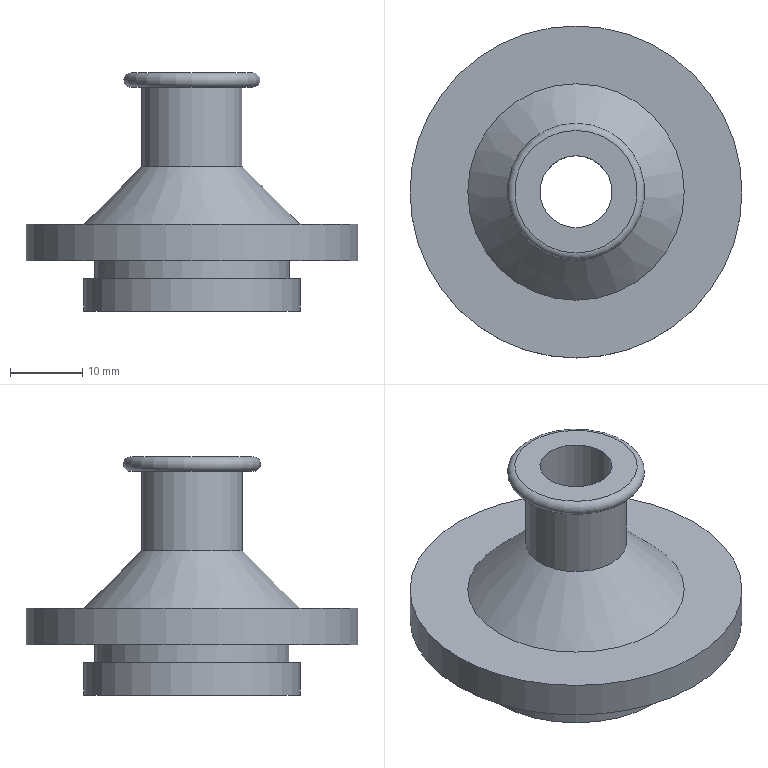Component | NX | LAMP_SOCKET | 1 solid | 15 faces | box 46 x 46 x 33 mm | volume 12206 mm3 | plane 7 | cylinder 6 | torus 1 | cone 1 | commonest cylinder face diameters 20 x1 10 x1 14 x1 46 x1 27 x1 30 x1
STEP:
#1=CARTESIAN_POINT('',(0.,0.,0.));
#2=DIRECTION('',(0.,0.,1.));
#3=DIRECTION('',(1.,0.,0.));
#4=AXIS2_PLACEMENT_3D('',#1,#2,#3);
#5=CARTESIAN_POINT('',(40.,-34.,89.));
#6=VERTEX_POINT('',#5);
#7=CARTESIAN_POINT('',(40.,-44.,89.));
#8=DIRECTION('',(0.,0.,-1.));
#9=DIRECTION('',(0.,1.,0.));
#10=AXIS2_PLACEMENT_3D('',#7,#8,#9);
#11=CIRCLE('',#10,10.);
#12=CARTESIAN_POINT('',(40.,-59.,89.));
#13=DIRECTION('',(0.,0.,1.));
#14=DIRECTION('',(0.,-1.,0.));
#15=AXIS2_PLACEMENT_3D('',#12,#13,#14);
#16=PLANE('',#15);
#17=CARTESIAN_POINT('',(-25.,0.));
#18=CARTESIAN_POINT('',(-25.,17.321));
#19=CARTESIAN_POINT('',(-10.,8.66));
#20=CARTESIAN_POINT('',(5.,0.));
#21=CARTESIAN_POINT('',(-10.,-8.66));
#22=CARTESIAN_POINT('',(-25.,-17.321));
#23=CARTESIAN_POINT('',(-25.,0.));
#24=(BOUNDED_CURVE()B_SPLINE_CURVE(2,(#17,#18,#19,#20,#21,#22,#23),.UNSPECIFIED.,.T.,.F.)B_SPLINE_CURVE_WITH_KNOTS((1,2,2,2,2,1),(-2.094,0.,2.094,4.189,6.283,8.378),.UNSPECIFIED.)CURVE()GEOMETRIC_REPRESENTATION_ITEM()RATIONAL_B_SPLINE_CURVE((1.,0.5,1.,0.5,1.,0.5,1.))REPRESENTATION_ITEM(''));
#25=(GEOMETRIC_REPRESENTATION_CONTEXT(2)PARAMETRIC_REPRESENTATION_CONTEXT()REPRESENTATION_CONTEXT('',''));
#26=DEFINITIONAL_REPRESENTATION('',(#24),#25);
#27=PCURVE('',#16,#26);
#28=CARTESIAN_POINT('',(40.,-44.,89.));
#29=DIRECTION('',(0.,0.,-1.));
#30=DIRECTION('',(0.,1.,0.));
#31=AXIS2_PLACEMENT_3D('',#28,#29,#30);
#32=CYLINDRICAL_SURFACE('',#31,10.);
#33=CARTESIAN_POINT('',(0.,0.));
#34=DIRECTION('',(1.,0.));
#35=VECTOR('',#34,1.);
#36=LINE('',#33,#35);
#37=(GEOMETRIC_REPRESENTATION_CONTEXT(2)PARAMETRIC_REPRESENTATION_CONTEXT()REPRESENTATION_CONTEXT('',''));
#38=DEFINITIONAL_REPRESENTATION('',(#36),#37);
#39=PCURVE('',#32,#38);
#40=SURFACE_CURVE('',#11,(#27,#39),.PCURVE_S1.);
#41=EDGE_CURVE('',#6,#6,#40,.T.);
#42=ORIENTED_EDGE('',*,*,#41,.F.);
#43=EDGE_LOOP('',(#42));
#44=FACE_BOUND('',#43,.T.);
#45=CARTESIAN_POINT('',(40.,-29.,89.));
#46=VERTEX_POINT('',#45);
#47=CARTESIAN_POINT('',(40.,-44.,89.));
#48=DIRECTION('',(0.,0.,-1.));
#49=DIRECTION('',(0.,1.,0.));
#50=AXIS2_PLACEMENT_3D('',#47,#48,#49);
#51=CIRCLE('',#50,15.);
#52=CARTESIAN_POINT('',(-30.,0.));
#53=CARTESIAN_POINT('',(-30.,25.981));
#54=CARTESIAN_POINT('',(-7.5,12.99));
#55=CARTESIAN_POINT('',(15.,0.));
#56=CARTESIAN_POINT('',(-7.5,-12.99));
#57=CARTESIAN_POINT('',(-30.,-25.981));
#58=CARTESIAN_POINT('',(-30.,0.));
#59=(BOUNDED_CURVE()B_SPLINE_CURVE(2,(#52,#53,#54,#55,#56,#57,#58),.UNSPECIFIED.,.T.,.F.)B_SPLINE_CURVE_WITH_KNOTS((1,2,2,2,2,1),(-2.094,0.,2.094,4.189,6.283,8.378),.UNSPECIFIED.)CURVE()GEOMETRIC_REPRESENTATION_ITEM()RATIONAL_B_SPLINE_CURVE((1.,0.5,1.,0.5,1.,0.5,1.))REPRESENTATION_ITEM(''));
#60=(GEOMETRIC_REPRESENTATION_CONTEXT(2)PARAMETRIC_REPRESENTATION_CONTEXT()REPRESENTATION_CONTEXT('',''));
#61=DEFINITIONAL_REPRESENTATION('',(#59),#60);
#62=PCURVE('',#16,#61);
#63=CARTESIAN_POINT('',(40.,-44.,89.));
#64=DIRECTION('',(0.,0.,-1.));
#65=DIRECTION('',(0.,1.,0.));
#66=AXIS2_PLACEMENT_3D('',#63,#64,#65);
#67=CYLINDRICAL_SURFACE('',#66,15.);
#68=CARTESIAN_POINT('',(0.,0.));
#69=DIRECTION('',(1.,0.));
#70=VECTOR('',#69,1.);
#71=LINE('',#68,#70);
#72=(GEOMETRIC_REPRESENTATION_CONTEXT(2)PARAMETRIC_REPRESENTATION_CONTEXT()REPRESENTATION_CONTEXT('',''));
#73=DEFINITIONAL_REPRESENTATION('',(#71),#72);
#74=PCURVE('',#67,#73);
#75=SURFACE_CURVE('',#51,(#62,#74),.PCURVE_S1.);
#76=EDGE_CURVE('',#46,#46,#75,.T.);
#77=ORIENTED_EDGE('',*,*,#76,.T.);
#78=EDGE_LOOP('',(#77));
#79=FACE_BOUND('',#78,.T.);
#80=ADVANCED_FACE('',(#44,#79),#16,.F.);
#81=CARTESIAN_POINT('',(40.,-34.,104.));
#82=VERTEX_POINT('',#81);
#83=CARTESIAN_POINT('',(40.,-44.,104.));
#84=DIRECTION('',(0.,0.,-1.));
#85=DIRECTION('',(0.,1.,0.));
#86=AXIS2_PLACEMENT_3D('',#83,#84,#85);
#87=CIRCLE('',#86,10.);
#88=CARTESIAN_POINT('',(0.,-15.));
#89=DIRECTION('',(1.,0.));
#90=VECTOR('',#89,1.);
#91=LINE('',#88,#90);
#92=(GEOMETRIC_REPRESENTATION_CONTEXT(2)PARAMETRIC_REPRESENTATION_CONTEXT()REPRESENTATION_CONTEXT('',''));
#93=DEFINITIONAL_REPRESENTATION('',(#91),#92);
#94=PCURVE('',#32,#93);
#95=CARTESIAN_POINT('',(40.,-54.,104.));
#96=DIRECTION('',(0.,0.,1.));
#97=DIRECTION('',(0.,-1.,0.));
#98=AXIS2_PLACEMENT_3D('',#95,#96,#97);
#99=PLANE('',#98);
#100=CARTESIAN_POINT('',(-20.,0.));
#101=CARTESIAN_POINT('',(-20.,17.321));
#102=CARTESIAN_POINT('',(-5.,8.66));
#103=CARTESIAN_POINT('',(10.,0.));
#104=CARTESIAN_POINT('',(-5.,-8.66));
#105=CARTESIAN_POINT('',(-20.,-17.321));
#106=CARTESIAN_POINT('',(-20.,0.));
#107=(BOUNDED_CURVE()B_SPLINE_CURVE(2,(#100,#101,#102,#103,#104,#105,#106),.UNSPECIFIED.,.T.,.F.)B_SPLINE_CURVE_WITH_KNOTS((1,2,2,2,2,1),(-2.094,0.,2.094,4.189,6.283,8.378),.UNSPECIFIED.)CURVE()GEOMETRIC_REPRESENTATION_ITEM()RATIONAL_B_SPLINE_CURVE((1.,0.5,1.,0.5,1.,0.5,1.))REPRESENTATION_ITEM(''));
#108=(GEOMETRIC_REPRESENTATION_CONTEXT(2)PARAMETRIC_REPRESENTATION_CONTEXT()REPRESENTATION_CONTEXT('',''));
#109=DEFINITIONAL_REPRESENTATION('',(#107),#108);
#110=PCURVE('',#99,#109);
#111=SURFACE_CURVE('',#87,(#94,#110),.PCURVE_S1.);
#112=EDGE_CURVE('',#82,#82,#111,.T.);
#113=ORIENTED_EDGE('',*,*,#112,.T.);
#114=CARTESIAN_POINT('',(40.,-34.,104.));
#115=CARTESIAN_POINT('',(40.,-34.,89.));
#116=B_SPLINE_CURVE_WITH_KNOTS('',1,(#114,#115),.UNSPECIFIED.,.F.,.F.,(2,2),(-15.,0.),.PIECEWISE_BEZIER_KNOTS.);
#117=CARTESIAN_POINT('',(6.283,0.));
#118=DIRECTION('',(0.,1.));
#119=VECTOR('',#118,1.);
#120=LINE('',#117,#119);
#121=(GEOMETRIC_REPRESENTATION_CONTEXT(2)PARAMETRIC_REPRESENTATION_CONTEXT()REPRESENTATION_CONTEXT('',''));
#122=DEFINITIONAL_REPRESENTATION('',(#120),#121);
#123=PCURVE('',#32,#122);
#124=CARTESIAN_POINT('',(0.,0.));
#125=DIRECTION('',(0.,1.));
#126=VECTOR('',#125,1.);
#127=LINE('',#124,#126);
#128=(GEOMETRIC_REPRESENTATION_CONTEXT(2)PARAMETRIC_REPRESENTATION_CONTEXT()REPRESENTATION_CONTEXT('',''));
#129=DEFINITIONAL_REPRESENTATION('',(#127),#128);
#130=PCURVE('',#32,#129);
#131=SEAM_CURVE('',#116,(#123,#130),.PCURVE_S1.);
#132=EDGE_CURVE('',#82,#6,#131,.T.);
#133=ORIENTED_EDGE('',*,*,#132,.T.);
#134=ORIENTED_EDGE('',*,*,#41,.F.);
#135=ORIENTED_EDGE('',*,*,#132,.F.);
#136=EDGE_LOOP('',(#113,#133,#134,#135));
#137=FACE_BOUND('',#136,.F.);
#138=ADVANCED_FACE('',(#137),#32,.F.);
#139=CARTESIAN_POINT('',(40.,-39.,104.));
#140=VERTEX_POINT('',#139);
#141=CARTESIAN_POINT('',(40.,-44.,104.));
#142=DIRECTION('',(0.,0.,-1.));
#143=DIRECTION('',(0.,1.,0.));
#144=AXIS2_PLACEMENT_3D('',#141,#142,#143);
#145=CIRCLE('',#144,5.);
#146=CARTESIAN_POINT('',(-15.,0.));
#147=CARTESIAN_POINT('',(-15.,8.66));
#148=CARTESIAN_POINT('',(-7.5,4.33));
#149=CARTESIAN_POINT('',(-0.,0.));
#150=CARTESIAN_POINT('',(-7.5,-4.33));
#151=CARTESIAN_POINT('',(-15.,-8.66));
#152=CARTESIAN_POINT('',(-15.,0.));
#153=(BOUNDED_CURVE()B_SPLINE_CURVE(2,(#146,#147,#148,#149,#150,#151,#152),.UNSPECIFIED.,.T.,.F.)B_SPLINE_CURVE_WITH_KNOTS((1,2,2,2,2,1),(-2.094,0.,2.094,4.189,6.283,8.378),.UNSPECIFIED.)CURVE()GEOMETRIC_REPRESENTATION_ITEM()RATIONAL_B_SPLINE_CURVE((1.,0.5,1.,0.5,1.,0.5,1.))REPRESENTATION_ITEM(''));
#154=(GEOMETRIC_REPRESENTATION_CONTEXT(2)PARAMETRIC_REPRESENTATION_CONTEXT()REPRESENTATION_CONTEXT('',''));
#155=DEFINITIONAL_REPRESENTATION('',(#153),#154);
#156=PCURVE('',#99,#155);
#157=CARTESIAN_POINT('',(40.,-44.,89.));
#158=DIRECTION('',(0.,0.,-1.));
#159=DIRECTION('',(0.,1.,0.));
#160=AXIS2_PLACEMENT_3D('',#157,#158,#159);
#161=CYLINDRICAL_SURFACE('',#160,5.);
#162=CARTESIAN_POINT('',(0.,-15.));
#163=DIRECTION('',(1.,0.));
#164=VECTOR('',#163,1.);
#165=LINE('',#162,#164);
#166=(GEOMETRIC_REPRESENTATION_CONTEXT(2)PARAMETRIC_REPRESENTATION_CONTEXT()REPRESENTATION_CONTEXT('',''));
#167=DEFINITIONAL_REPRESENTATION('',(#165),#166);
#168=PCURVE('',#161,#167);
#169=SURFACE_CURVE('',#145,(#156,#168),.PCURVE_S1.);
#170=EDGE_CURVE('',#140,#140,#169,.T.);
#171=ORIENTED_EDGE('',*,*,#170,.F.);
#172=EDGE_LOOP('',(#171));
#173=FACE_BOUND('',#172,.T.);
#174=ORIENTED_EDGE('',*,*,#112,.T.);
#175=EDGE_LOOP('',(#174));
#176=FACE_BOUND('',#175,.T.);
#177=ADVANCED_FACE('',(#173,#176),#99,.F.);
#178=CARTESIAN_POINT('',(40.,-39.,122.));
#179=VERTEX_POINT('',#178);
#180=CARTESIAN_POINT('',(40.,-44.,122.));
#181=DIRECTION('',(0.,0.,-1.));
#182=DIRECTION('',(0.,1.,0.));
#183=AXIS2_PLACEMENT_3D('',#180,#181,#182);
#184=CIRCLE('',#183,5.);
#185=CARTESIAN_POINT('',(0.,-33.));
#186=DIRECTION('',(1.,0.));
#187=VECTOR('',#186,1.);
#188=LINE('',#185,#187);
#189=(GEOMETRIC_REPRESENTATION_CONTEXT(2)PARAMETRIC_REPRESENTATION_CONTEXT()REPRESENTATION_CONTEXT('',''));
#190=DEFINITIONAL_REPRESENTATION('',(#188),#189);
#191=PCURVE('',#161,#190);
#192=CARTESIAN_POINT('',(40.,-49.,122.));
#193=DIRECTION('',(0.,0.,-1.));
#194=DIRECTION('',(0.,1.,0.));
#195=AXIS2_PLACEMENT_3D('',#192,#193,#194);
#196=PLANE('',#195);
#197=CARTESIAN_POINT('',(5.,0.));
#198=DIRECTION('',(1.,0.));
#199=AXIS2_PLACEMENT_2D('',#197,#198);
#200=CIRCLE('',#199,5.);
#201=(GEOMETRIC_REPRESENTATION_CONTEXT(2)PARAMETRIC_REPRESENTATION_CONTEXT()REPRESENTATION_CONTEXT('',''));
#202=DEFINITIONAL_REPRESENTATION('',(#200),#201);
#203=PCURVE('',#196,#202);
#204=SURFACE_CURVE('',#184,(#191,#203),.PCURVE_S1.);
#205=EDGE_CURVE('',#179,#179,#204,.T.);
#206=ORIENTED_EDGE('',*,*,#205,.T.);
#207=CARTESIAN_POINT('',(40.,-39.,122.));
#208=CARTESIAN_POINT('',(40.,-39.,104.));
#209=B_SPLINE_CURVE_WITH_KNOTS('',1,(#207,#208),.UNSPECIFIED.,.F.,.F.,(2,2),(-33.,-15.),.PIECEWISE_BEZIER_KNOTS.);
#210=CARTESIAN_POINT('',(6.283,0.));
#211=DIRECTION('',(0.,1.));
#212=VECTOR('',#211,1.);
#213=LINE('',#210,#212);
#214=(GEOMETRIC_REPRESENTATION_CONTEXT(2)PARAMETRIC_REPRESENTATION_CONTEXT()REPRESENTATION_CONTEXT('',''));
#215=DEFINITIONAL_REPRESENTATION('',(#213),#214);
#216=PCURVE('',#161,#215);
#217=CARTESIAN_POINT('',(0.,0.));
#218=DIRECTION('',(0.,1.));
#219=VECTOR('',#218,1.);
#220=LINE('',#217,#219);
#221=(GEOMETRIC_REPRESENTATION_CONTEXT(2)PARAMETRIC_REPRESENTATION_CONTEXT()REPRESENTATION_CONTEXT('',''));
#222=DEFINITIONAL_REPRESENTATION('',(#220),#221);
#223=PCURVE('',#161,#222);
#224=SEAM_CURVE('',#209,(#216,#223),.PCURVE_S1.);
#225=EDGE_CURVE('',#179,#140,#224,.T.);
#226=ORIENTED_EDGE('',*,*,#225,.T.);
#227=ORIENTED_EDGE('',*,*,#170,.F.);
#228=ORIENTED_EDGE('',*,*,#225,.F.);
#229=EDGE_LOOP('',(#206,#226,#227,#228));
#230=FACE_BOUND('',#229,.F.);
#231=ADVANCED_FACE('',(#230),#161,.F.);
#232=CARTESIAN_POINT('',(40.,-35.5,122.));
#233=VERTEX_POINT('',#232);
#234=CARTESIAN_POINT('',(40.,-44.,122.));
#235=DIRECTION('',(0.,0.,-1.));
#236=DIRECTION('',(0.,1.,0.));
#237=AXIS2_PLACEMENT_3D('',#234,#235,#236);
#238=CIRCLE('',#237,8.5);
#239=CARTESIAN_POINT('',(5.,0.));
#240=DIRECTION('',(1.,0.));
#241=AXIS2_PLACEMENT_2D('',#239,#240);
#242=CIRCLE('',#241,8.5);
#243=(GEOMETRIC_REPRESENTATION_CONTEXT(2)PARAMETRIC_REPRESENTATION_CONTEXT()REPRESENTATION_CONTEXT('',''));
#244=DEFINITIONAL_REPRESENTATION('',(#242),#243);
#245=PCURVE('',#196,#244);
#246=CARTESIAN_POINT('',(40.,-44.,121.));
#247=DIRECTION('',(0.,0.,-1.));
#248=DIRECTION('',(0.,1.,0.));
#249=AXIS2_PLACEMENT_3D('',#246,#247,#248);
#250=TOROIDAL_SURFACE('',#249,8.5,1.);
#251=CARTESIAN_POINT('',(0.,4.712));
#252=DIRECTION('',(1.,0.));
#253=VECTOR('',#252,1.);
#254=LINE('',#251,#253);
#255=(GEOMETRIC_REPRESENTATION_CONTEXT(2)PARAMETRIC_REPRESENTATION_CONTEXT()REPRESENTATION_CONTEXT('',''));
#256=DEFINITIONAL_REPRESENTATION('',(#254),#255);
#257=PCURVE('',#250,#256);
#258=SURFACE_CURVE('',#238,(#245,#257),.PCURVE_S1.);
#259=EDGE_CURVE('',#233,#233,#258,.T.);
#260=ORIENTED_EDGE('',*,*,#259,.F.);
#261=EDGE_LOOP('',(#260));
#262=FACE_BOUND('',#261,.T.);
#263=ORIENTED_EDGE('',*,*,#205,.T.);
#264=EDGE_LOOP('',(#263));
#265=FACE_BOUND('',#264,.T.);
#266=ADVANCED_FACE('',(#262,#265),#196,.F.);
#267=CARTESIAN_POINT('',(40.,-35.5,120.));
#268=VERTEX_POINT('',#267);
#269=CARTESIAN_POINT('',(40.,-44.,120.));
#270=DIRECTION('',(0.,0.,-1.));
#271=DIRECTION('',(0.,1.,0.));
#272=AXIS2_PLACEMENT_3D('',#269,#270,#271);
#273=CIRCLE('',#272,8.5);
#274=CARTESIAN_POINT('',(0.,7.854));
#275=DIRECTION('',(1.,0.));
#276=VECTOR('',#275,1.);
#277=LINE('',#274,#276);
#278=(GEOMETRIC_REPRESENTATION_CONTEXT(2)PARAMETRIC_REPRESENTATION_CONTEXT()REPRESENTATION_CONTEXT('',''));
#279=DEFINITIONAL_REPRESENTATION('',(#277),#278);
#280=PCURVE('',#250,#279);
#281=CARTESIAN_POINT('',(40.,-52.5,120.));
#282=DIRECTION('',(0.,0.,1.));
#283=DIRECTION('',(0.,-1.,0.));
#284=AXIS2_PLACEMENT_3D('',#281,#282,#283);
#285=PLANE('',#284);
#286=CARTESIAN_POINT('',(-17.,0.));
#287=CARTESIAN_POINT('',(-17.,14.722));
#288=CARTESIAN_POINT('',(-4.25,7.361));
#289=CARTESIAN_POINT('',(8.5,0.));
#290=CARTESIAN_POINT('',(-4.25,-7.361));
#291=CARTESIAN_POINT('',(-17.,-14.722));
#292=CARTESIAN_POINT('',(-17.,0.));
#293=(BOUNDED_CURVE()B_SPLINE_CURVE(2,(#286,#287,#288,#289,#290,#291,#292),.UNSPECIFIED.,.T.,.F.)B_SPLINE_CURVE_WITH_KNOTS((1,2,2,2,2,1),(-2.094,0.,2.094,4.189,6.283,8.378),.UNSPECIFIED.)CURVE()GEOMETRIC_REPRESENTATION_ITEM()RATIONAL_B_SPLINE_CURVE((1.,0.5,1.,0.5,1.,0.5,1.))REPRESENTATION_ITEM(''));
#294=(GEOMETRIC_REPRESENTATION_CONTEXT(2)PARAMETRIC_REPRESENTATION_CONTEXT()REPRESENTATION_CONTEXT('',''));
#295=DEFINITIONAL_REPRESENTATION('',(#293),#294);
#296=PCURVE('',#285,#295);
#297=SURFACE_CURVE('',#273,(#280,#296),.PCURVE_S1.);
#298=EDGE_CURVE('',#268,#268,#297,.T.);
#299=ORIENTED_EDGE('',*,*,#298,.F.);
#300=CARTESIAN_POINT('',(40.,-35.5,122.));
#301=CARTESIAN_POINT('',(40.,-35.107,122.));
#302=CARTESIAN_POINT('',(40.,-34.715,121.824));
#303=CARTESIAN_POINT('',(40.,-34.414,121.471));
#304=CARTESIAN_POINT('',(40.,-34.298,121.));
#305=CARTESIAN_POINT('',(40.,-34.414,120.529));
#306=CARTESIAN_POINT('',(40.,-34.715,120.176));
#307=CARTESIAN_POINT('',(40.,-35.107,120.));
#308=CARTESIAN_POINT('',(40.,-35.5,120.));
#309=B_SPLINE_CURVE_WITH_KNOTS('',8,(#300,#301,#302,#303,#304,#305,#306,#307,#308),.UNSPECIFIED.,.F.,.F.,(9,9),(-1.571,1.571),.PIECEWISE_BEZIER_KNOTS.);
#310=CARTESIAN_POINT('',(0.,6.283));
#311=DIRECTION('',(0.,1.));
#312=VECTOR('',#311,1.);
#313=LINE('',#310,#312);
#314=(GEOMETRIC_REPRESENTATION_CONTEXT(2)PARAMETRIC_REPRESENTATION_CONTEXT()REPRESENTATION_CONTEXT('',''));
#315=DEFINITIONAL_REPRESENTATION('',(#313),#314);
#316=PCURVE('',#250,#315);
#317=CARTESIAN_POINT('',(6.283,6.283));
#318=DIRECTION('',(0.,1.));
#319=VECTOR('',#318,1.);
#320=LINE('',#317,#319);
#321=(GEOMETRIC_REPRESENTATION_CONTEXT(2)PARAMETRIC_REPRESENTATION_CONTEXT()REPRESENTATION_CONTEXT('',''));
#322=DEFINITIONAL_REPRESENTATION('',(#320),#321);
#323=PCURVE('',#250,#322);
#324=SEAM_CURVE('',#309,(#316,#323),.PCURVE_S1.);
#325=EDGE_CURVE('',#233,#268,#324,.T.);
#326=ORIENTED_EDGE('',*,*,#325,.F.);
#327=ORIENTED_EDGE('',*,*,#259,.T.);
#328=ORIENTED_EDGE('',*,*,#325,.T.);
#329=EDGE_LOOP('',(#299,#326,#327,#328));
#330=FACE_BOUND('',#329,.T.);
#331=ADVANCED_FACE('',(#330),#250,.T.);
#332=CARTESIAN_POINT('',(40.,-37.,120.));
#333=VERTEX_POINT('',#332);
#334=CARTESIAN_POINT('',(40.,-44.,120.));
#335=DIRECTION('',(0.,0.,-1.));
#336=DIRECTION('',(0.,1.,0.));
#337=AXIS2_PLACEMENT_3D('',#334,#335,#336);
#338=CIRCLE('',#337,7.);
#339=CARTESIAN_POINT('',(-15.5,0.));
#340=CARTESIAN_POINT('',(-15.5,12.124));
#341=CARTESIAN_POINT('',(-5.,6.062));
#342=CARTESIAN_POINT('',(5.5,0.));
#343=CARTESIAN_POINT('',(-5.,-6.062));
#344=CARTESIAN_POINT('',(-15.5,-12.124));
#345=CARTESIAN_POINT('',(-15.5,0.));
#346=(BOUNDED_CURVE()B_SPLINE_CURVE(2,(#339,#340,#341,#342,#343,#344,#345),.UNSPECIFIED.,.T.,.F.)B_SPLINE_CURVE_WITH_KNOTS((1,2,2,2,2,1),(-2.094,0.,2.094,4.189,6.283,8.378),.UNSPECIFIED.)CURVE()GEOMETRIC_REPRESENTATION_ITEM()RATIONAL_B_SPLINE_CURVE((1.,0.5,1.,0.5,1.,0.5,1.))REPRESENTATION_ITEM(''));
#347=(GEOMETRIC_REPRESENTATION_CONTEXT(2)PARAMETRIC_REPRESENTATION_CONTEXT()REPRESENTATION_CONTEXT('',''));
#348=DEFINITIONAL_REPRESENTATION('',(#346),#347);
#349=PCURVE('',#285,#348);
#350=CARTESIAN_POINT('',(40.,-44.,89.));
#351=DIRECTION('',(0.,0.,-1.));
#352=DIRECTION('',(0.,1.,0.));
#353=AXIS2_PLACEMENT_3D('',#350,#351,#352);
#354=CYLINDRICAL_SURFACE('',#353,7.);
#355=CARTESIAN_POINT('',(0.,-31.));
#356=DIRECTION('',(1.,0.));
#357=VECTOR('',#356,1.);
#358=LINE('',#355,#357);
#359=(GEOMETRIC_REPRESENTATION_CONTEXT(2)PARAMETRIC_REPRESENTATION_CONTEXT()REPRESENTATION_CONTEXT('',''));
#360=DEFINITIONAL_REPRESENTATION('',(#358),#359);
#361=PCURVE('',#354,#360);
#362=SURFACE_CURVE('',#338,(#349,#361),.PCURVE_S1.);
#363=EDGE_CURVE('',#333,#333,#362,.T.);
#364=ORIENTED_EDGE('',*,*,#363,.F.);
#365=EDGE_LOOP('',(#364));
#366=FACE_BOUND('',#365,.T.);
#367=ORIENTED_EDGE('',*,*,#298,.T.);
#368=EDGE_LOOP('',(#367));
#369=FACE_BOUND('',#368,.T.);
#370=ADVANCED_FACE('',(#366,#369),#285,.F.);
#371=CARTESIAN_POINT('',(40.,-37.,109.));
#372=VERTEX_POINT('',#371);
#373=CARTESIAN_POINT('',(40.,-44.,109.));
#374=DIRECTION('',(0.,0.,-1.));
#375=DIRECTION('',(0.,1.,0.));
#376=AXIS2_PLACEMENT_3D('',#373,#374,#375);
#377=CIRCLE('',#376,7.);
#378=CARTESIAN_POINT('',(0.,-20.));
#379=DIRECTION('',(1.,0.));
#380=VECTOR('',#379,1.);
#381=LINE('',#378,#380);
#382=(GEOMETRIC_REPRESENTATION_CONTEXT(2)PARAMETRIC_REPRESENTATION_CONTEXT()REPRESENTATION_CONTEXT('',''));
#383=DEFINITIONAL_REPRESENTATION('',(#381),#382);
#384=PCURVE('',#354,#383);
#385=CARTESIAN_POINT('',(40.,-44.,109.));
#386=DIRECTION('',(0.,0.,-1.));
#387=DIRECTION('',(0.,1.,0.));
#388=AXIS2_PLACEMENT_3D('',#385,#386,#387);
#389=CONICAL_SURFACE('',#388,7.,0.7854);
#390=CARTESIAN_POINT('',(0.,0.));
#391=DIRECTION('',(1.,0.));
#392=VECTOR('',#391,1.);
#393=LINE('',#390,#392);
#394=(GEOMETRIC_REPRESENTATION_CONTEXT(2)PARAMETRIC_REPRESENTATION_CONTEXT()REPRESENTATION_CONTEXT('',''));
#395=DEFINITIONAL_REPRESENTATION('',(#393),#394);
#396=PCURVE('',#389,#395);
#397=SURFACE_CURVE('',#377,(#384,#396),.PCURVE_S1.);
#398=EDGE_CURVE('',#372,#372,#397,.T.);
#399=ORIENTED_EDGE('',*,*,#398,.F.);
#400=CARTESIAN_POINT('',(40.,-37.,120.));
#401=CARTESIAN_POINT('',(40.,-37.,109.));
#402=B_SPLINE_CURVE_WITH_KNOTS('',1,(#400,#401),.UNSPECIFIED.,.F.,.F.,(2,2),(-31.,-20.),.PIECEWISE_BEZIER_KNOTS.);
#403=CARTESIAN_POINT('',(0.,0.));
#404=DIRECTION('',(0.,1.));
#405=VECTOR('',#404,1.);
#406=LINE('',#403,#405);
#407=(GEOMETRIC_REPRESENTATION_CONTEXT(2)PARAMETRIC_REPRESENTATION_CONTEXT()REPRESENTATION_CONTEXT('',''));
#408=DEFINITIONAL_REPRESENTATION('',(#406),#407);
#409=PCURVE('',#354,#408);
#410=CARTESIAN_POINT('',(6.283,0.));
#411=DIRECTION('',(0.,1.));
#412=VECTOR('',#411,1.);
#413=LINE('',#410,#412);
#414=(GEOMETRIC_REPRESENTATION_CONTEXT(2)PARAMETRIC_REPRESENTATION_CONTEXT()REPRESENTATION_CONTEXT('',''));
#415=DEFINITIONAL_REPRESENTATION('',(#413),#414);
#416=PCURVE('',#354,#415);
#417=SEAM_CURVE('',#402,(#409,#416),.PCURVE_S1.);
#418=EDGE_CURVE('',#333,#372,#417,.T.);
#419=ORIENTED_EDGE('',*,*,#418,.F.);
#420=ORIENTED_EDGE('',*,*,#363,.T.);
#421=ORIENTED_EDGE('',*,*,#418,.T.);
#422=EDGE_LOOP('',(#399,#419,#420,#421));
#423=FACE_BOUND('',#422,.T.);
#424=ADVANCED_FACE('',(#423),#354,.T.);
#425=CARTESIAN_POINT('',(40.,-29.,101.));
#426=VERTEX_POINT('',#425);
#427=CARTESIAN_POINT('',(40.,-44.,101.));
#428=DIRECTION('',(0.,0.,-1.));
#429=DIRECTION('',(0.,1.,0.));
#430=AXIS2_PLACEMENT_3D('',#427,#428,#429);
#431=CIRCLE('',#430,15.);
#432=CARTESIAN_POINT('',(0.,8.));
#433=DIRECTION('',(1.,0.));
#434=VECTOR('',#433,1.);
#435=LINE('',#432,#434);
#436=(GEOMETRIC_REPRESENTATION_CONTEXT(2)PARAMETRIC_REPRESENTATION_CONTEXT()REPRESENTATION_CONTEXT('',''));
#437=DEFINITIONAL_REPRESENTATION('',(#435),#436);
#438=PCURVE('',#389,#437);
#439=CARTESIAN_POINT('',(40.,-59.,101.));
#440=DIRECTION('',(0.,0.,-1.));
#441=DIRECTION('',(0.,1.,0.));
#442=AXIS2_PLACEMENT_3D('',#439,#440,#441);
#443=PLANE('',#442);
#444=CARTESIAN_POINT('',(15.,0.));
#445=DIRECTION('',(1.,0.));
#446=AXIS2_PLACEMENT_2D('',#444,#445);
#447=CIRCLE('',#446,15.);
#448=(GEOMETRIC_REPRESENTATION_CONTEXT(2)PARAMETRIC_REPRESENTATION_CONTEXT()REPRESENTATION_CONTEXT('',''));
#449=DEFINITIONAL_REPRESENTATION('',(#447),#448);
#450=PCURVE('',#443,#449);
#451=SURFACE_CURVE('',#431,(#438,#450),.PCURVE_S1.);
#452=EDGE_CURVE('',#426,#426,#451,.T.);
#453=ORIENTED_EDGE('',*,*,#452,.F.);
#454=CARTESIAN_POINT('',(40.,-37.,109.));
#455=CARTESIAN_POINT('',(40.,-29.,101.));
#456=B_SPLINE_CURVE_WITH_KNOTS('',1,(#454,#455),.UNSPECIFIED.,.F.,.F.,(2,2),(0.,11.314),.PIECEWISE_BEZIER_KNOTS.);
#457=CARTESIAN_POINT('',(0.,0.));
#458=DIRECTION('',(0.,1.));
#459=VECTOR('',#458,1.);
#460=LINE('',#457,#459);
#461=(GEOMETRIC_REPRESENTATION_CONTEXT(2)PARAMETRIC_REPRESENTATION_CONTEXT()REPRESENTATION_CONTEXT('',''));
#462=DEFINITIONAL_REPRESENTATION('',(#460),#461);
#463=PCURVE('',#389,#462);
#464=CARTESIAN_POINT('',(6.283,0.));
#465=DIRECTION('',(0.,1.));
#466=VECTOR('',#465,1.);
#467=LINE('',#464,#466);
#468=(GEOMETRIC_REPRESENTATION_CONTEXT(2)PARAMETRIC_REPRESENTATION_CONTEXT()REPRESENTATION_CONTEXT('',''));
#469=DEFINITIONAL_REPRESENTATION('',(#467),#468);
#470=PCURVE('',#389,#469);
#471=SEAM_CURVE('',#456,(#463,#470),.PCURVE_S1.);
#472=EDGE_CURVE('',#372,#426,#471,.T.);
#473=ORIENTED_EDGE('',*,*,#472,.F.);
#474=ORIENTED_EDGE('',*,*,#398,.T.);
#475=ORIENTED_EDGE('',*,*,#472,.T.);
#476=EDGE_LOOP('',(#453,#473,#474,#475));
#477=FACE_BOUND('',#476,.T.);
#478=ADVANCED_FACE('',(#477),#389,.T.);
#479=CARTESIAN_POINT('',(40.,-21.,101.));
#480=VERTEX_POINT('',#479);
#481=CARTESIAN_POINT('',(40.,-44.,101.));
#482=DIRECTION('',(0.,0.,-1.));
#483=DIRECTION('',(0.,1.,0.));
#484=AXIS2_PLACEMENT_3D('',#481,#482,#483);
#485=CIRCLE('',#484,23.);
#486=CARTESIAN_POINT('',(15.,0.));
#487=DIRECTION('',(1.,0.));
#488=AXIS2_PLACEMENT_2D('',#486,#487);
#489=CIRCLE('',#488,23.);
#490=(GEOMETRIC_REPRESENTATION_CONTEXT(2)PARAMETRIC_REPRESENTATION_CONTEXT()REPRESENTATION_CONTEXT('',''));
#491=DEFINITIONAL_REPRESENTATION('',(#489),#490);
#492=PCURVE('',#443,#491);
#493=CARTESIAN_POINT('',(40.,-44.,89.));
#494=DIRECTION('',(0.,0.,-1.));
#495=DIRECTION('',(0.,1.,0.));
#496=AXIS2_PLACEMENT_3D('',#493,#494,#495);
#497=CYLINDRICAL_SURFACE('',#496,23.);
#498=CARTESIAN_POINT('',(0.,-12.));
#499=DIRECTION('',(1.,0.));
#500=VECTOR('',#499,1.);
#501=LINE('',#498,#500);
#502=(GEOMETRIC_REPRESENTATION_CONTEXT(2)PARAMETRIC_REPRESENTATION_CONTEXT()REPRESENTATION_CONTEXT('',''));
#503=DEFINITIONAL_REPRESENTATION('',(#501),#502);
#504=PCURVE('',#497,#503);
#505=SURFACE_CURVE('',#485,(#492,#504),.PCURVE_S1.);
#506=EDGE_CURVE('',#480,#480,#505,.T.);
#507=ORIENTED_EDGE('',*,*,#506,.F.);
#508=EDGE_LOOP('',(#507));
#509=FACE_BOUND('',#508,.T.);
#510=ORIENTED_EDGE('',*,*,#452,.T.);
#511=EDGE_LOOP('',(#510));
#512=FACE_BOUND('',#511,.T.);
#513=ADVANCED_FACE('',(#509,#512),#443,.F.);
#514=CARTESIAN_POINT('',(40.,-21.,96.));
#515=VERTEX_POINT('',#514);
#516=CARTESIAN_POINT('',(40.,-44.,96.));
#517=DIRECTION('',(0.,0.,-1.));
#518=DIRECTION('',(0.,1.,0.));
#519=AXIS2_PLACEMENT_3D('',#516,#517,#518);
#520=CIRCLE('',#519,23.);
#521=CARTESIAN_POINT('',(0.,-7.));
#522=DIRECTION('',(1.,0.));
#523=VECTOR('',#522,1.);
#524=LINE('',#521,#523);
#525=(GEOMETRIC_REPRESENTATION_CONTEXT(2)PARAMETRIC_REPRESENTATION_CONTEXT()REPRESENTATION_CONTEXT('',''));
#526=DEFINITIONAL_REPRESENTATION('',(#524),#525);
#527=PCURVE('',#497,#526);
#528=CARTESIAN_POINT('',(40.,-67.,96.));
#529=DIRECTION('',(0.,0.,1.));
#530=DIRECTION('',(0.,-1.,0.));
#531=AXIS2_PLACEMENT_3D('',#528,#529,#530);
#532=PLANE('',#531);
#533=CARTESIAN_POINT('',(-46.,0.));
#534=CARTESIAN_POINT('',(-46.,39.837));
#535=CARTESIAN_POINT('',(-11.5,19.919));
#536=CARTESIAN_POINT('',(23.,0.));
#537=CARTESIAN_POINT('',(-11.5,-19.919));
#538=CARTESIAN_POINT('',(-46.,-39.837));
#539=CARTESIAN_POINT('',(-46.,0.));
#540=(BOUNDED_CURVE()B_SPLINE_CURVE(2,(#533,#534,#535,#536,#537,#538,#539),.UNSPECIFIED.,.T.,.F.)B_SPLINE_CURVE_WITH_KNOTS((1,2,2,2,2,1),(-2.094,0.,2.094,4.189,6.283,8.378),.UNSPECIFIED.)CURVE()GEOMETRIC_REPRESENTATION_ITEM()RATIONAL_B_SPLINE_CURVE((1.,0.5,1.,0.5,1.,0.5,1.))REPRESENTATION_ITEM(''));
#541=(GEOMETRIC_REPRESENTATION_CONTEXT(2)PARAMETRIC_REPRESENTATION_CONTEXT()REPRESENTATION_CONTEXT('',''));
#542=DEFINITIONAL_REPRESENTATION('',(#540),#541);
#543=PCURVE('',#532,#542);
#544=SURFACE_CURVE('',#520,(#527,#543),.PCURVE_S1.);
#545=EDGE_CURVE('',#515,#515,#544,.T.);
#546=ORIENTED_EDGE('',*,*,#545,.F.);
#547=CARTESIAN_POINT('',(40.,-21.,101.));
#548=CARTESIAN_POINT('',(40.,-21.,96.));
#549=B_SPLINE_CURVE_WITH_KNOTS('',1,(#547,#548),.UNSPECIFIED.,.F.,.F.,(2,2),(-12.,-7.),.PIECEWISE_BEZIER_KNOTS.);
#550=CARTESIAN_POINT('',(0.,0.));
#551=DIRECTION('',(0.,1.));
#552=VECTOR('',#551,1.);
#553=LINE('',#550,#552);
#554=(GEOMETRIC_REPRESENTATION_CONTEXT(2)PARAMETRIC_REPRESENTATION_CONTEXT()REPRESENTATION_CONTEXT('',''));
#555=DEFINITIONAL_REPRESENTATION('',(#553),#554);
#556=PCURVE('',#497,#555);
#557=CARTESIAN_POINT('',(6.283,0.));
#558=DIRECTION('',(0.,1.));
#559=VECTOR('',#558,1.);
#560=LINE('',#557,#559);
#561=(GEOMETRIC_REPRESENTATION_CONTEXT(2)PARAMETRIC_REPRESENTATION_CONTEXT()REPRESENTATION_CONTEXT('',''));
#562=DEFINITIONAL_REPRESENTATION('',(#560),#561);
#563=PCURVE('',#497,#562);
#564=SEAM_CURVE('',#549,(#556,#563),.PCURVE_S1.);
#565=EDGE_CURVE('',#480,#515,#564,.T.);
#566=ORIENTED_EDGE('',*,*,#565,.F.);
#567=ORIENTED_EDGE('',*,*,#506,.T.);
#568=ORIENTED_EDGE('',*,*,#565,.T.);
#569=EDGE_LOOP('',(#546,#566,#567,#568));
#570=FACE_BOUND('',#569,.T.);
#571=ADVANCED_FACE('',(#570),#497,.T.);
#572=CARTESIAN_POINT('',(40.,-30.5,96.));
#573=VERTEX_POINT('',#572);
#574=CARTESIAN_POINT('',(40.,-44.,96.));
#575=DIRECTION('',(0.,0.,-1.));
#576=DIRECTION('',(0.,1.,0.));
#577=AXIS2_PLACEMENT_3D('',#574,#575,#576);
#578=CIRCLE('',#577,13.5);
#579=CARTESIAN_POINT('',(-36.5,0.));
#580=CARTESIAN_POINT('',(-36.5,23.383));
#581=CARTESIAN_POINT('',(-16.25,11.691));
#582=CARTESIAN_POINT('',(4.,0.));
#583=CARTESIAN_POINT('',(-16.25,-11.691));
#584=CARTESIAN_POINT('',(-36.5,-23.383));
#585=CARTESIAN_POINT('',(-36.5,0.));
#586=(BOUNDED_CURVE()B_SPLINE_CURVE(2,(#579,#580,#581,#582,#583,#584,#585),.UNSPECIFIED.,.T.,.F.)B_SPLINE_CURVE_WITH_KNOTS((1,2,2,2,2,1),(-2.094,0.,2.094,4.189,6.283,8.378),.UNSPECIFIED.)CURVE()GEOMETRIC_REPRESENTATION_ITEM()RATIONAL_B_SPLINE_CURVE((1.,0.5,1.,0.5,1.,0.5,1.))REPRESENTATION_ITEM(''));
#587=(GEOMETRIC_REPRESENTATION_CONTEXT(2)PARAMETRIC_REPRESENTATION_CONTEXT()REPRESENTATION_CONTEXT('',''));
#588=DEFINITIONAL_REPRESENTATION('',(#586),#587);
#589=PCURVE('',#532,#588);
#590=CARTESIAN_POINT('',(40.,-44.,89.));
#591=DIRECTION('',(0.,0.,-1.));
#592=DIRECTION('',(0.,1.,0.));
#593=AXIS2_PLACEMENT_3D('',#590,#591,#592);
#594=CYLINDRICAL_SURFACE('',#593,13.5);
#595=CARTESIAN_POINT('',(0.,-7.));
#596=DIRECTION('',(1.,0.));
#597=VECTOR('',#596,1.);
#598=LINE('',#595,#597);
#599=(GEOMETRIC_REPRESENTATION_CONTEXT(2)PARAMETRIC_REPRESENTATION_CONTEXT()REPRESENTATION_CONTEXT('',''));
#600=DEFINITIONAL_REPRESENTATION('',(#598),#599);
#601=PCURVE('',#594,#600);
#602=SURFACE_CURVE('',#578,(#589,#601),.PCURVE_S1.);
#603=EDGE_CURVE('',#573,#573,#602,.T.);
#604=ORIENTED_EDGE('',*,*,#603,.F.);
#605=EDGE_LOOP('',(#604));
#606=FACE_BOUND('',#605,.T.);
#607=ORIENTED_EDGE('',*,*,#545,.T.);
#608=EDGE_LOOP('',(#607));
#609=FACE_BOUND('',#608,.T.);
#610=ADVANCED_FACE('',(#606,#609),#532,.F.);
#611=CARTESIAN_POINT('',(40.,-30.5,93.5));
#612=VERTEX_POINT('',#611);
#613=CARTESIAN_POINT('',(40.,-44.,93.5));
#614=DIRECTION('',(0.,0.,-1.));
#615=DIRECTION('',(0.,1.,0.));
#616=AXIS2_PLACEMENT_3D('',#613,#614,#615);
#617=CIRCLE('',#616,13.5);
#618=CARTESIAN_POINT('',(0.,-4.5));
#619=DIRECTION('',(1.,0.));
#620=VECTOR('',#619,1.);
#621=LINE('',#618,#620);
#622=(GEOMETRIC_REPRESENTATION_CONTEXT(2)PARAMETRIC_REPRESENTATION_CONTEXT()REPRESENTATION_CONTEXT('',''));
#623=DEFINITIONAL_REPRESENTATION('',(#621),#622);
#624=PCURVE('',#594,#623);
#625=CARTESIAN_POINT('',(40.,-57.5,93.5));
#626=DIRECTION('',(0.,0.,-1.));
#627=DIRECTION('',(0.,1.,0.));
#628=AXIS2_PLACEMENT_3D('',#625,#626,#627);
#629=PLANE('',#628);
#630=CARTESIAN_POINT('',(13.5,0.));
#631=DIRECTION('',(1.,0.));
#632=AXIS2_PLACEMENT_2D('',#630,#631);
#633=CIRCLE('',#632,13.5);
#634=(GEOMETRIC_REPRESENTATION_CONTEXT(2)PARAMETRIC_REPRESENTATION_CONTEXT()REPRESENTATION_CONTEXT('',''));
#635=DEFINITIONAL_REPRESENTATION('',(#633),#634);
#636=PCURVE('',#629,#635);
#637=SURFACE_CURVE('',#617,(#624,#636),.PCURVE_S1.);
#638=EDGE_CURVE('',#612,#612,#637,.T.);
#639=ORIENTED_EDGE('',*,*,#638,.F.);
#640=CARTESIAN_POINT('',(40.,-30.5,96.));
#641=CARTESIAN_POINT('',(40.,-30.5,93.5));
#642=B_SPLINE_CURVE_WITH_KNOTS('',1,(#640,#641),.UNSPECIFIED.,.F.,.F.,(2,2),(-7.,-4.5),.PIECEWISE_BEZIER_KNOTS.);
#643=CARTESIAN_POINT('',(0.,0.));
#644=DIRECTION('',(0.,1.));
#645=VECTOR('',#644,1.);
#646=LINE('',#643,#645);
#647=(GEOMETRIC_REPRESENTATION_CONTEXT(2)PARAMETRIC_REPRESENTATION_CONTEXT()REPRESENTATION_CONTEXT('',''));
#648=DEFINITIONAL_REPRESENTATION('',(#646),#647);
#649=PCURVE('',#594,#648);
#650=CARTESIAN_POINT('',(6.283,0.));
#651=DIRECTION('',(0.,1.));
#652=VECTOR('',#651,1.);
#653=LINE('',#650,#652);
#654=(GEOMETRIC_REPRESENTATION_CONTEXT(2)PARAMETRIC_REPRESENTATION_CONTEXT()REPRESENTATION_CONTEXT('',''));
#655=DEFINITIONAL_REPRESENTATION('',(#653),#654);
#656=PCURVE('',#594,#655);
#657=SEAM_CURVE('',#642,(#649,#656),.PCURVE_S1.);
#658=EDGE_CURVE('',#573,#612,#657,.T.);
#659=ORIENTED_EDGE('',*,*,#658,.F.);
#660=ORIENTED_EDGE('',*,*,#603,.T.);
#661=ORIENTED_EDGE('',*,*,#658,.T.);
#662=EDGE_LOOP('',(#639,#659,#660,#661));
#663=FACE_BOUND('',#662,.T.);
#664=ADVANCED_FACE('',(#663),#594,.T.);
#665=CARTESIAN_POINT('',(40.,-29.,93.5));
#666=VERTEX_POINT('',#665);
#667=CARTESIAN_POINT('',(40.,-44.,93.5));
#668=DIRECTION('',(0.,0.,-1.));
#669=DIRECTION('',(0.,1.,0.));
#670=AXIS2_PLACEMENT_3D('',#667,#668,#669);
#671=CIRCLE('',#670,15.);
#672=CARTESIAN_POINT('',(13.5,0.));
#673=DIRECTION('',(1.,0.));
#674=AXIS2_PLACEMENT_2D('',#672,#673);
#675=CIRCLE('',#674,15.);
#676=(GEOMETRIC_REPRESENTATION_CONTEXT(2)PARAMETRIC_REPRESENTATION_CONTEXT()REPRESENTATION_CONTEXT('',''));
#677=DEFINITIONAL_REPRESENTATION('',(#675),#676);
#678=PCURVE('',#629,#677);
#679=CARTESIAN_POINT('',(0.,-4.5));
#680=DIRECTION('',(1.,0.));
#681=VECTOR('',#680,1.);
#682=LINE('',#679,#681);
#683=(GEOMETRIC_REPRESENTATION_CONTEXT(2)PARAMETRIC_REPRESENTATION_CONTEXT()REPRESENTATION_CONTEXT('',''));
#684=DEFINITIONAL_REPRESENTATION('',(#682),#683);
#685=PCURVE('',#67,#684);
#686=SURFACE_CURVE('',#671,(#678,#685),.PCURVE_S1.);
#687=EDGE_CURVE('',#666,#666,#686,.T.);
#688=ORIENTED_EDGE('',*,*,#687,.F.);
#689=EDGE_LOOP('',(#688));
#690=FACE_BOUND('',#689,.T.);
#691=ORIENTED_EDGE('',*,*,#638,.T.);
#692=EDGE_LOOP('',(#691));
#693=FACE_BOUND('',#692,.T.);
#694=ADVANCED_FACE('',(#690,#693),#629,.F.);
#695=ORIENTED_EDGE('',*,*,#76,.F.);
#696=CARTESIAN_POINT('',(40.,-29.,93.5));
#697=CARTESIAN_POINT('',(40.,-29.,89.));
#698=B_SPLINE_CURVE_WITH_KNOTS('',1,(#696,#697),.UNSPECIFIED.,.F.,.F.,(2,2),(-4.5,0.),.PIECEWISE_BEZIER_KNOTS.);
#699=CARTESIAN_POINT('',(0.,0.));
#700=DIRECTION('',(0.,1.));
#701=VECTOR('',#700,1.);
#702=LINE('',#699,#701);
#703=(GEOMETRIC_REPRESENTATION_CONTEXT(2)PARAMETRIC_REPRESENTATION_CONTEXT()REPRESENTATION_CONTEXT('',''));
#704=DEFINITIONAL_REPRESENTATION('',(#702),#703);
#705=PCURVE('',#67,#704);
#706=CARTESIAN_POINT('',(6.283,0.));
#707=DIRECTION('',(0.,1.));
#708=VECTOR('',#707,1.);
#709=LINE('',#706,#708);
#710=(GEOMETRIC_REPRESENTATION_CONTEXT(2)PARAMETRIC_REPRESENTATION_CONTEXT()REPRESENTATION_CONTEXT('',''));
#711=DEFINITIONAL_REPRESENTATION('',(#709),#710);
#712=PCURVE('',#67,#711);
#713=SEAM_CURVE('',#698,(#705,#712),.PCURVE_S1.);
#714=EDGE_CURVE('',#666,#46,#713,.T.);
#715=ORIENTED_EDGE('',*,*,#714,.F.);
#716=ORIENTED_EDGE('',*,*,#687,.T.);
#717=ORIENTED_EDGE('',*,*,#714,.T.);
#718=EDGE_LOOP('',(#695,#715,#716,#717));
#719=FACE_BOUND('',#718,.T.);
#720=ADVANCED_FACE('',(#719),#67,.T.);
#721=CLOSED_SHELL('',(#80,#138,#177,#231,#266,#331,#370,#424,#478,#513,#571,#610,#664,#694,#720));
#722=MANIFOLD_SOLID_BREP('',#721);
#723=(LENGTH_UNIT()NAMED_UNIT(*)SI_UNIT(.MILLI.,.METRE.));
#724=UNCERTAINTY_MEASURE_WITH_UNIT(LENGTH_MEASURE(0.00001),#723,'','');
#725=(NAMED_UNIT(*)PLANE_ANGLE_UNIT()SI_UNIT($,.RADIAN.));
#726=(NAMED_UNIT(*)SI_UNIT($,.STERADIAN.)SOLID_ANGLE_UNIT());
#727=(GEOMETRIC_REPRESENTATION_CONTEXT(3)GLOBAL_UNCERTAINTY_ASSIGNED_CONTEXT((#724))GLOBAL_UNIT_ASSIGNED_CONTEXT((#723,#725,#726))REPRESENTATION_CONTEXT('',''));
#728=ADVANCED_BREP_SHAPE_REPRESENTATION('',(#4,#722),#727);